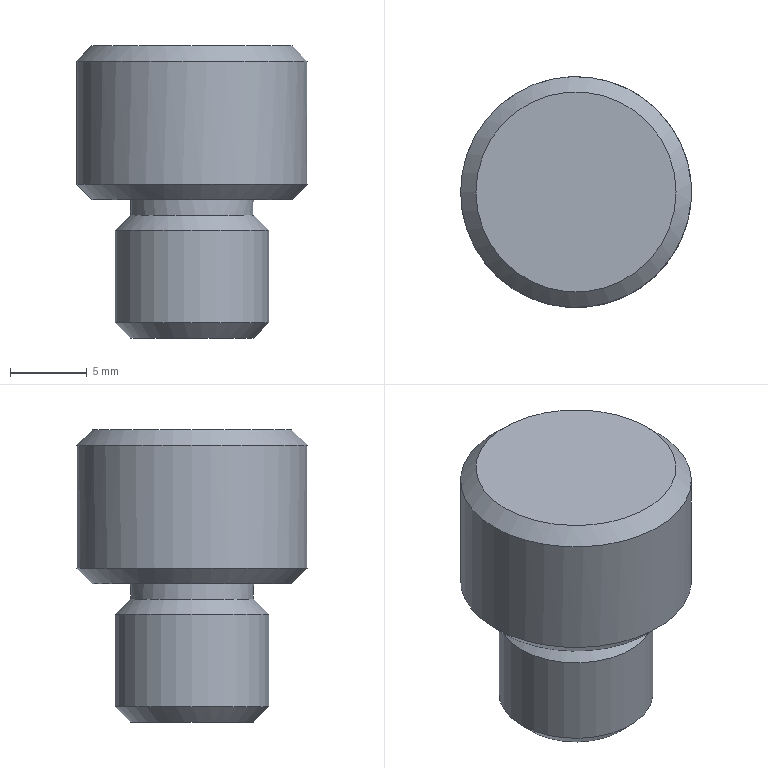Component | NX | SUPPORT_PIN | 1 solid | 10 faces | box 15 x 15 x 19 mm | volume 2371 mm3 | cone 4 | plane 3 | cylinder 3 | commonest cylinder face diameters 10 x1 8 x1 15 x1
STEP:
#1=CARTESIAN_POINT('',(0.,0.,0.));
#2=DIRECTION('',(0.,0.,1.));
#3=DIRECTION('',(1.,0.,0.));
#4=AXIS2_PLACEMENT_3D('',#1,#2,#3);
#5=CARTESIAN_POINT('',(-68.5,126.,81.));
#6=VERTEX_POINT('',#5);
#7=CARTESIAN_POINT('',(-72.5,126.,81.));
#8=DIRECTION('',(0.,0.,-1.));
#9=DIRECTION('',(1.,0.,0.));
#10=AXIS2_PLACEMENT_3D('',#7,#8,#9);
#11=CIRCLE('',#10,4.);
#12=CARTESIAN_POINT('',(-72.5,126.,81.));
#13=DIRECTION('',(0.,0.,-1.));
#14=DIRECTION('',(1.,0.,0.));
#15=AXIS2_PLACEMENT_3D('',#12,#13,#14);
#16=PLANE('',#15);
#17=CARTESIAN_POINT('',(0.,0.));
#18=DIRECTION('',(1.,0.));
#19=AXIS2_PLACEMENT_2D('',#17,#18);
#20=CIRCLE('',#19,4.);
#21=(GEOMETRIC_REPRESENTATION_CONTEXT(2)PARAMETRIC_REPRESENTATION_CONTEXT()REPRESENTATION_CONTEXT('',''));
#22=DEFINITIONAL_REPRESENTATION('',(#20),#21);
#23=PCURVE('',#16,#22);
#24=CARTESIAN_POINT('',(-72.5,126.,82.));
#25=DIRECTION('',(0.,0.,1.));
#26=DIRECTION('',(-1.,0.,0.));
#27=AXIS2_PLACEMENT_3D('',#24,#25,#26);
#28=CONICAL_SURFACE('',#27,5.,0.7854);
#29=CARTESIAN_POINT('',(9.425,-1.));
#30=DIRECTION('',(-1.,0.));
#31=VECTOR('',#30,1.);
#32=LINE('',#29,#31);
#33=(GEOMETRIC_REPRESENTATION_CONTEXT(2)PARAMETRIC_REPRESENTATION_CONTEXT()REPRESENTATION_CONTEXT('',''));
#34=DEFINITIONAL_REPRESENTATION('',(#32),#33);
#35=PCURVE('',#28,#34);
#36=SURFACE_CURVE('',#11,(#23,#35),.PCURVE_S1.);
#37=EDGE_CURVE('',#6,#6,#36,.T.);
#38=ORIENTED_EDGE('',*,*,#37,.T.);
#39=EDGE_LOOP('',(#38));
#40=FACE_BOUND('',#39,.T.);
#41=ADVANCED_FACE('',(#40),#16,.T.);
#42=CARTESIAN_POINT('',(-67.5,126.,82.));
#43=VERTEX_POINT('',#42);
#44=CARTESIAN_POINT('',(-77.5,126.,82.));
#45=VERTEX_POINT('',#44);
#46=CARTESIAN_POINT('',(-72.5,126.,82.));
#47=DIRECTION('',(0.,0.,1.));
#48=DIRECTION('',(1.,0.,0.));
#49=AXIS2_PLACEMENT_3D('',#46,#47,#48);
#50=CIRCLE('',#49,5.);
#51=CARTESIAN_POINT('',(-72.5,126.,81.));
#52=DIRECTION('',(0.,0.,1.));
#53=DIRECTION('',(-1.,0.,0.));
#54=AXIS2_PLACEMENT_3D('',#51,#52,#53);
#55=CYLINDRICAL_SURFACE('',#54,5.);
#56=CARTESIAN_POINT('',(3.142,1.));
#57=DIRECTION('',(1.,0.));
#58=VECTOR('',#57,1.);
#59=LINE('',#56,#58);
#60=(GEOMETRIC_REPRESENTATION_CONTEXT(2)PARAMETRIC_REPRESENTATION_CONTEXT()REPRESENTATION_CONTEXT('',''));
#61=DEFINITIONAL_REPRESENTATION('',(#59),#60);
#62=PCURVE('',#55,#61);
#63=CARTESIAN_POINT('',(3.142,0.));
#64=DIRECTION('',(1.,0.));
#65=VECTOR('',#64,1.);
#66=LINE('',#63,#65);
#67=(GEOMETRIC_REPRESENTATION_CONTEXT(2)PARAMETRIC_REPRESENTATION_CONTEXT()REPRESENTATION_CONTEXT('',''));
#68=DEFINITIONAL_REPRESENTATION('',(#66),#67);
#69=PCURVE('',#28,#68);
#70=SURFACE_CURVE('',#50,(#62,#69),.PCURVE_S1.);
#71=EDGE_CURVE('',#43,#45,#70,.T.);
#72=ORIENTED_EDGE('',*,*,#71,.T.);
#73=CARTESIAN_POINT('',(-77.5,126.,88.));
#74=VERTEX_POINT('',#73);
#75=CARTESIAN_POINT('',(-77.5,126.,82.));
#76=CARTESIAN_POINT('',(-77.5,126.,88.));
#77=B_SPLINE_CURVE_WITH_KNOTS('',1,(#75,#76),.UNSPECIFIED.,.F.,.F.,(2,2),(1.,7.),.PIECEWISE_BEZIER_KNOTS.);
#78=CARTESIAN_POINT('',(6.283,0.));
#79=DIRECTION('',(0.,1.));
#80=VECTOR('',#79,1.);
#81=LINE('',#78,#80);
#82=(GEOMETRIC_REPRESENTATION_CONTEXT(2)PARAMETRIC_REPRESENTATION_CONTEXT()REPRESENTATION_CONTEXT('',''));
#83=DEFINITIONAL_REPRESENTATION('',(#81),#82);
#84=PCURVE('',#55,#83);
#85=CARTESIAN_POINT('',(0.,0.));
#86=DIRECTION('',(0.,1.));
#87=VECTOR('',#86,1.);
#88=LINE('',#85,#87);
#89=(GEOMETRIC_REPRESENTATION_CONTEXT(2)PARAMETRIC_REPRESENTATION_CONTEXT()REPRESENTATION_CONTEXT('',''));
#90=DEFINITIONAL_REPRESENTATION('',(#88),#89);
#91=PCURVE('',#55,#90);
#92=SEAM_CURVE('',#77,(#84,#91),.PCURVE_S1.);
#93=EDGE_CURVE('',#45,#74,#92,.T.);
#94=ORIENTED_EDGE('',*,*,#93,.T.);
#95=CARTESIAN_POINT('',(-72.5,126.,88.));
#96=DIRECTION('',(0.,0.,-1.));
#97=DIRECTION('',(-1.,0.,0.));
#98=AXIS2_PLACEMENT_3D('',#95,#96,#97);
#99=CIRCLE('',#98,5.);
#100=CARTESIAN_POINT('',(6.283,7.));
#101=DIRECTION('',(-1.,0.));
#102=VECTOR('',#101,1.);
#103=LINE('',#100,#102);
#104=(GEOMETRIC_REPRESENTATION_CONTEXT(2)PARAMETRIC_REPRESENTATION_CONTEXT()REPRESENTATION_CONTEXT('',''));
#105=DEFINITIONAL_REPRESENTATION('',(#103),#104);
#106=PCURVE('',#55,#105);
#107=CARTESIAN_POINT('',(-72.5,126.,88.));
#108=DIRECTION('',(0.,0.,-1.));
#109=DIRECTION('',(1.,0.,0.));
#110=AXIS2_PLACEMENT_3D('',#107,#108,#109);
#111=CONICAL_SURFACE('',#110,5.,0.7854);
#112=CARTESIAN_POINT('',(3.142,0.));
#113=DIRECTION('',(1.,0.));
#114=VECTOR('',#113,1.);
#115=LINE('',#112,#114);
#116=(GEOMETRIC_REPRESENTATION_CONTEXT(2)PARAMETRIC_REPRESENTATION_CONTEXT()REPRESENTATION_CONTEXT('',''));
#117=DEFINITIONAL_REPRESENTATION('',(#115),#116);
#118=PCURVE('',#111,#117);
#119=SURFACE_CURVE('',#99,(#106,#118),.PCURVE_S1.);
#120=EDGE_CURVE('',#74,#74,#119,.T.);
#121=ORIENTED_EDGE('',*,*,#120,.T.);
#122=ORIENTED_EDGE('',*,*,#93,.F.);
#123=CARTESIAN_POINT('',(-72.5,126.,82.));
#124=DIRECTION('',(0.,0.,1.));
#125=DIRECTION('',(1.,0.,0.));
#126=AXIS2_PLACEMENT_3D('',#123,#124,#125);
#127=CIRCLE('',#126,5.);
#128=CARTESIAN_POINT('',(-3.142,1.));
#129=DIRECTION('',(1.,0.));
#130=VECTOR('',#129,1.);
#131=LINE('',#128,#130);
#132=(GEOMETRIC_REPRESENTATION_CONTEXT(2)PARAMETRIC_REPRESENTATION_CONTEXT()REPRESENTATION_CONTEXT('',''));
#133=DEFINITIONAL_REPRESENTATION('',(#131),#132);
#134=PCURVE('',#55,#133);
#135=CARTESIAN_POINT('',(3.142,0.));
#136=DIRECTION('',(1.,0.));
#137=VECTOR('',#136,1.);
#138=LINE('',#135,#137);
#139=(GEOMETRIC_REPRESENTATION_CONTEXT(2)PARAMETRIC_REPRESENTATION_CONTEXT()REPRESENTATION_CONTEXT('',''));
#140=DEFINITIONAL_REPRESENTATION('',(#138),#139);
#141=PCURVE('',#28,#140);
#142=SURFACE_CURVE('',#127,(#134,#141),.PCURVE_S1.);
#143=EDGE_CURVE('',#45,#43,#142,.T.);
#144=ORIENTED_EDGE('',*,*,#143,.T.);
#145=EDGE_LOOP('',(#72,#94,#121,#122,#144));
#146=FACE_BOUND('',#145,.T.);
#147=ADVANCED_FACE('',(#146),#55,.T.);
#148=CARTESIAN_POINT('',(-76.5,126.,90.));
#149=VERTEX_POINT('',#148);
#150=CARTESIAN_POINT('',(-68.5,126.,90.));
#151=VERTEX_POINT('',#150);
#152=CARTESIAN_POINT('',(-72.5,126.,90.));
#153=DIRECTION('',(0.,0.,1.));
#154=DIRECTION('',(1.,0.,0.));
#155=AXIS2_PLACEMENT_3D('',#152,#153,#154);
#156=CIRCLE('',#155,4.);
#157=CARTESIAN_POINT('',(-72.5,126.,89.));
#158=DIRECTION('',(0.,0.,1.));
#159=DIRECTION('',(-1.,0.,0.));
#160=AXIS2_PLACEMENT_3D('',#157,#158,#159);
#161=CYLINDRICAL_SURFACE('',#160,4.);
#162=CARTESIAN_POINT('',(-3.142,1.));
#163=DIRECTION('',(1.,0.));
#164=VECTOR('',#163,1.);
#165=LINE('',#162,#164);
#166=(GEOMETRIC_REPRESENTATION_CONTEXT(2)PARAMETRIC_REPRESENTATION_CONTEXT()REPRESENTATION_CONTEXT('',''));
#167=DEFINITIONAL_REPRESENTATION('',(#165),#166);
#168=PCURVE('',#161,#167);
#169=CARTESIAN_POINT('',(-72.5,126.,90.));
#170=DIRECTION('',(0.,0.,-1.));
#171=DIRECTION('',(1.,0.,0.));
#172=AXIS2_PLACEMENT_3D('',#169,#170,#171);
#173=PLANE('',#172);
#174=CARTESIAN_POINT('',(4.,0.));
#175=CARTESIAN_POINT('',(4.,-6.928));
#176=CARTESIAN_POINT('',(-2.,-3.464));
#177=CARTESIAN_POINT('',(-8.,-0.));
#178=CARTESIAN_POINT('',(-2.,3.464));
#179=CARTESIAN_POINT('',(4.,6.928));
#180=CARTESIAN_POINT('',(4.,0.));
#181=(BOUNDED_CURVE()B_SPLINE_CURVE(2,(#174,#175,#176,#177,#178,#179,#180),.UNSPECIFIED.,.T.,.F.)B_SPLINE_CURVE_WITH_KNOTS((1,2,2,2,2,1),(-2.094,0.,2.094,4.189,6.283,8.378),.UNSPECIFIED.)CURVE()GEOMETRIC_REPRESENTATION_ITEM()RATIONAL_B_SPLINE_CURVE((1.,0.5,1.,0.5,1.,0.5,1.))REPRESENTATION_ITEM(''));
#182=(GEOMETRIC_REPRESENTATION_CONTEXT(2)PARAMETRIC_REPRESENTATION_CONTEXT()REPRESENTATION_CONTEXT('',''));
#183=DEFINITIONAL_REPRESENTATION('',(#181),#182);
#184=PCURVE('',#173,#183);
#185=SURFACE_CURVE('',#156,(#168,#184),.PCURVE_S1.);
#186=EDGE_CURVE('',#149,#151,#185,.T.);
#187=ORIENTED_EDGE('',*,*,#186,.F.);
#188=CARTESIAN_POINT('',(-76.5,126.,89.));
#189=VERTEX_POINT('',#188);
#190=CARTESIAN_POINT('',(-76.5,126.,89.));
#191=CARTESIAN_POINT('',(-76.5,126.,90.));
#192=B_SPLINE_CURVE_WITH_KNOTS('',1,(#190,#191),.UNSPECIFIED.,.F.,.F.,(2,2),(0.,1.),.PIECEWISE_BEZIER_KNOTS.);
#193=CARTESIAN_POINT('',(0.,0.));
#194=DIRECTION('',(0.,1.));
#195=VECTOR('',#194,1.);
#196=LINE('',#193,#195);
#197=(GEOMETRIC_REPRESENTATION_CONTEXT(2)PARAMETRIC_REPRESENTATION_CONTEXT()REPRESENTATION_CONTEXT('',''));
#198=DEFINITIONAL_REPRESENTATION('',(#196),#197);
#199=PCURVE('',#161,#198);
#200=CARTESIAN_POINT('',(6.283,0.));
#201=DIRECTION('',(0.,1.));
#202=VECTOR('',#201,1.);
#203=LINE('',#200,#202);
#204=(GEOMETRIC_REPRESENTATION_CONTEXT(2)PARAMETRIC_REPRESENTATION_CONTEXT()REPRESENTATION_CONTEXT('',''));
#205=DEFINITIONAL_REPRESENTATION('',(#203),#204);
#206=PCURVE('',#161,#205);
#207=SEAM_CURVE('',#192,(#199,#206),.PCURVE_S1.);
#208=EDGE_CURVE('',#189,#149,#207,.T.);
#209=ORIENTED_EDGE('',*,*,#208,.F.);
#210=CARTESIAN_POINT('',(-72.5,126.,89.));
#211=DIRECTION('',(0.,0.,1.));
#212=DIRECTION('',(-1.,0.,0.));
#213=AXIS2_PLACEMENT_3D('',#210,#211,#212);
#214=CIRCLE('',#213,4.);
#215=CARTESIAN_POINT('',(0.,0.));
#216=DIRECTION('',(1.,0.));
#217=VECTOR('',#216,1.);
#218=LINE('',#215,#217);
#219=(GEOMETRIC_REPRESENTATION_CONTEXT(2)PARAMETRIC_REPRESENTATION_CONTEXT()REPRESENTATION_CONTEXT('',''));
#220=DEFINITIONAL_REPRESENTATION('',(#218),#219);
#221=PCURVE('',#161,#220);
#222=CARTESIAN_POINT('',(9.425,-1.));
#223=DIRECTION('',(-1.,0.));
#224=VECTOR('',#223,1.);
#225=LINE('',#222,#224);
#226=(GEOMETRIC_REPRESENTATION_CONTEXT(2)PARAMETRIC_REPRESENTATION_CONTEXT()REPRESENTATION_CONTEXT('',''));
#227=DEFINITIONAL_REPRESENTATION('',(#225),#226);
#228=PCURVE('',#111,#227);
#229=SURFACE_CURVE('',#214,(#221,#228),.PCURVE_S1.);
#230=EDGE_CURVE('',#189,#189,#229,.T.);
#231=ORIENTED_EDGE('',*,*,#230,.T.);
#232=ORIENTED_EDGE('',*,*,#208,.T.);
#233=CARTESIAN_POINT('',(-72.5,126.,90.));
#234=DIRECTION('',(0.,0.,1.));
#235=DIRECTION('',(1.,0.,0.));
#236=AXIS2_PLACEMENT_3D('',#233,#234,#235);
#237=CIRCLE('',#236,4.);
#238=CARTESIAN_POINT('',(3.142,1.));
#239=DIRECTION('',(1.,0.));
#240=VECTOR('',#239,1.);
#241=LINE('',#238,#240);
#242=(GEOMETRIC_REPRESENTATION_CONTEXT(2)PARAMETRIC_REPRESENTATION_CONTEXT()REPRESENTATION_CONTEXT('',''));
#243=DEFINITIONAL_REPRESENTATION('',(#241),#242);
#244=PCURVE('',#161,#243);
#245=CARTESIAN_POINT('',(4.,0.));
#246=CARTESIAN_POINT('',(4.,-6.928));
#247=CARTESIAN_POINT('',(-2.,-3.464));
#248=CARTESIAN_POINT('',(-8.,-0.));
#249=CARTESIAN_POINT('',(-2.,3.464));
#250=CARTESIAN_POINT('',(4.,6.928));
#251=CARTESIAN_POINT('',(4.,0.));
#252=(BOUNDED_CURVE()B_SPLINE_CURVE(2,(#245,#246,#247,#248,#249,#250,#251),.UNSPECIFIED.,.T.,.F.)B_SPLINE_CURVE_WITH_KNOTS((1,2,2,2,2,1),(-2.094,0.,2.094,4.189,6.283,8.378),.UNSPECIFIED.)CURVE()GEOMETRIC_REPRESENTATION_ITEM()RATIONAL_B_SPLINE_CURVE((1.,0.5,1.,0.5,1.,0.5,1.))REPRESENTATION_ITEM(''));
#253=(GEOMETRIC_REPRESENTATION_CONTEXT(2)PARAMETRIC_REPRESENTATION_CONTEXT()REPRESENTATION_CONTEXT('',''));
#254=DEFINITIONAL_REPRESENTATION('',(#252),#253);
#255=PCURVE('',#173,#254);
#256=SURFACE_CURVE('',#237,(#244,#255),.PCURVE_S1.);
#257=EDGE_CURVE('',#151,#149,#256,.T.);
#258=ORIENTED_EDGE('',*,*,#257,.F.);
#259=EDGE_LOOP('',(#187,#209,#231,#232,#258));
#260=FACE_BOUND('',#259,.T.);
#261=ADVANCED_FACE('',(#260),#161,.T.);
#262=CARTESIAN_POINT('',(-79.,126.,100.));
#263=VERTEX_POINT('',#262);
#264=CARTESIAN_POINT('',(-72.5,126.,100.));
#265=DIRECTION('',(0.,0.,1.));
#266=DIRECTION('',(-1.,0.,0.));
#267=AXIS2_PLACEMENT_3D('',#264,#265,#266);
#268=CIRCLE('',#267,6.5);
#269=CARTESIAN_POINT('',(-72.5,126.,100.));
#270=DIRECTION('',(0.,0.,1.));
#271=DIRECTION('',(-1.,0.,0.));
#272=AXIS2_PLACEMENT_3D('',#269,#270,#271);
#273=PLANE('',#272);
#274=CARTESIAN_POINT('',(0.,0.));
#275=DIRECTION('',(1.,0.));
#276=AXIS2_PLACEMENT_2D('',#274,#275);
#277=CIRCLE('',#276,6.5);
#278=(GEOMETRIC_REPRESENTATION_CONTEXT(2)PARAMETRIC_REPRESENTATION_CONTEXT()REPRESENTATION_CONTEXT('',''));
#279=DEFINITIONAL_REPRESENTATION('',(#277),#278);
#280=PCURVE('',#273,#279);
#281=CARTESIAN_POINT('',(-72.5,126.,99.));
#282=DIRECTION('',(0.,0.,-1.));
#283=DIRECTION('',(1.,0.,0.));
#284=AXIS2_PLACEMENT_3D('',#281,#282,#283);
#285=CONICAL_SURFACE('',#284,7.5,0.7854);
#286=CARTESIAN_POINT('',(9.425,-1.));
#287=DIRECTION('',(-1.,0.));
#288=VECTOR('',#287,1.);
#289=LINE('',#286,#288);
#290=(GEOMETRIC_REPRESENTATION_CONTEXT(2)PARAMETRIC_REPRESENTATION_CONTEXT()REPRESENTATION_CONTEXT('',''));
#291=DEFINITIONAL_REPRESENTATION('',(#289),#290);
#292=PCURVE('',#285,#291);
#293=SURFACE_CURVE('',#268,(#280,#292),.PCURVE_S1.);
#294=EDGE_CURVE('',#263,#263,#293,.T.);
#295=ORIENTED_EDGE('',*,*,#294,.T.);
#296=EDGE_LOOP('',(#295));
#297=FACE_BOUND('',#296,.T.);
#298=ADVANCED_FACE('',(#297),#273,.T.);
#299=CARTESIAN_POINT('',(-66.,126.,90.));
#300=VERTEX_POINT('',#299);
#301=CARTESIAN_POINT('',(-72.5,126.,90.));
#302=DIRECTION('',(0.,0.,-1.));
#303=DIRECTION('',(1.,0.,0.));
#304=AXIS2_PLACEMENT_3D('',#301,#302,#303);
#305=CIRCLE('',#304,6.5);
#306=CARTESIAN_POINT('',(0.,0.));
#307=DIRECTION('',(1.,0.));
#308=AXIS2_PLACEMENT_2D('',#306,#307);
#309=CIRCLE('',#308,6.5);
#310=(GEOMETRIC_REPRESENTATION_CONTEXT(2)PARAMETRIC_REPRESENTATION_CONTEXT()REPRESENTATION_CONTEXT('',''));
#311=DEFINITIONAL_REPRESENTATION('',(#309),#310);
#312=PCURVE('',#173,#311);
#313=CARTESIAN_POINT('',(-72.5,126.,91.));
#314=DIRECTION('',(0.,0.,1.));
#315=DIRECTION('',(-1.,0.,0.));
#316=AXIS2_PLACEMENT_3D('',#313,#314,#315);
#317=CONICAL_SURFACE('',#316,7.5,0.7854);
#318=CARTESIAN_POINT('',(9.425,-1.));
#319=DIRECTION('',(-1.,0.));
#320=VECTOR('',#319,1.);
#321=LINE('',#318,#320);
#322=(GEOMETRIC_REPRESENTATION_CONTEXT(2)PARAMETRIC_REPRESENTATION_CONTEXT()REPRESENTATION_CONTEXT('',''));
#323=DEFINITIONAL_REPRESENTATION('',(#321),#322);
#324=PCURVE('',#317,#323);
#325=SURFACE_CURVE('',#305,(#312,#324),.PCURVE_S1.);
#326=EDGE_CURVE('',#300,#300,#325,.T.);
#327=ORIENTED_EDGE('',*,*,#326,.T.);
#328=EDGE_LOOP('',(#327));
#329=FACE_BOUND('',#328,.T.);
#330=ORIENTED_EDGE('',*,*,#257,.T.);
#331=ORIENTED_EDGE('',*,*,#186,.T.);
#332=EDGE_LOOP('',(#330,#331));
#333=FACE_BOUND('',#332,.T.);
#334=ADVANCED_FACE('',(#329,#333),#173,.T.);
#335=CARTESIAN_POINT('',(-65.,126.,91.));
#336=VERTEX_POINT('',#335);
#337=CARTESIAN_POINT('',(-80.,126.,91.));
#338=VERTEX_POINT('',#337);
#339=CARTESIAN_POINT('',(-72.5,126.,91.));
#340=DIRECTION('',(0.,0.,1.));
#341=DIRECTION('',(1.,0.,0.));
#342=AXIS2_PLACEMENT_3D('',#339,#340,#341);
#343=CIRCLE('',#342,7.5);
#344=CARTESIAN_POINT('',(-72.5,126.,90.));
#345=DIRECTION('',(0.,0.,1.));
#346=DIRECTION('',(-1.,0.,0.));
#347=AXIS2_PLACEMENT_3D('',#344,#345,#346);
#348=CYLINDRICAL_SURFACE('',#347,7.5);
#349=CARTESIAN_POINT('',(3.142,1.));
#350=DIRECTION('',(1.,0.));
#351=VECTOR('',#350,1.);
#352=LINE('',#349,#351);
#353=(GEOMETRIC_REPRESENTATION_CONTEXT(2)PARAMETRIC_REPRESENTATION_CONTEXT()REPRESENTATION_CONTEXT('',''));
#354=DEFINITIONAL_REPRESENTATION('',(#352),#353);
#355=PCURVE('',#348,#354);
#356=CARTESIAN_POINT('',(3.142,0.));
#357=DIRECTION('',(1.,0.));
#358=VECTOR('',#357,1.);
#359=LINE('',#356,#358);
#360=(GEOMETRIC_REPRESENTATION_CONTEXT(2)PARAMETRIC_REPRESENTATION_CONTEXT()REPRESENTATION_CONTEXT('',''));
#361=DEFINITIONAL_REPRESENTATION('',(#359),#360);
#362=PCURVE('',#317,#361);
#363=SURFACE_CURVE('',#343,(#355,#362),.PCURVE_S1.);
#364=EDGE_CURVE('',#336,#338,#363,.T.);
#365=ORIENTED_EDGE('',*,*,#364,.T.);
#366=CARTESIAN_POINT('',(-80.,126.,99.));
#367=VERTEX_POINT('',#366);
#368=CARTESIAN_POINT('',(-80.,126.,91.));
#369=CARTESIAN_POINT('',(-80.,126.,99.));
#370=B_SPLINE_CURVE_WITH_KNOTS('',1,(#368,#369),.UNSPECIFIED.,.F.,.F.,(2,2),(1.,9.),.PIECEWISE_BEZIER_KNOTS.);
#371=CARTESIAN_POINT('',(6.283,0.));
#372=DIRECTION('',(0.,1.));
#373=VECTOR('',#372,1.);
#374=LINE('',#371,#373);
#375=(GEOMETRIC_REPRESENTATION_CONTEXT(2)PARAMETRIC_REPRESENTATION_CONTEXT()REPRESENTATION_CONTEXT('',''));
#376=DEFINITIONAL_REPRESENTATION('',(#374),#375);
#377=PCURVE('',#348,#376);
#378=CARTESIAN_POINT('',(0.,0.));
#379=DIRECTION('',(0.,1.));
#380=VECTOR('',#379,1.);
#381=LINE('',#378,#380);
#382=(GEOMETRIC_REPRESENTATION_CONTEXT(2)PARAMETRIC_REPRESENTATION_CONTEXT()REPRESENTATION_CONTEXT('',''));
#383=DEFINITIONAL_REPRESENTATION('',(#381),#382);
#384=PCURVE('',#348,#383);
#385=SEAM_CURVE('',#370,(#377,#384),.PCURVE_S1.);
#386=EDGE_CURVE('',#338,#367,#385,.T.);
#387=ORIENTED_EDGE('',*,*,#386,.T.);
#388=CARTESIAN_POINT('',(-72.5,126.,99.));
#389=DIRECTION('',(0.,0.,-1.));
#390=DIRECTION('',(-1.,0.,0.));
#391=AXIS2_PLACEMENT_3D('',#388,#389,#390);
#392=CIRCLE('',#391,7.5);
#393=CARTESIAN_POINT('',(6.283,9.));
#394=DIRECTION('',(-1.,0.));
#395=VECTOR('',#394,1.);
#396=LINE('',#393,#395);
#397=(GEOMETRIC_REPRESENTATION_CONTEXT(2)PARAMETRIC_REPRESENTATION_CONTEXT()REPRESENTATION_CONTEXT('',''));
#398=DEFINITIONAL_REPRESENTATION('',(#396),#397);
#399=PCURVE('',#348,#398);
#400=CARTESIAN_POINT('',(3.142,0.));
#401=DIRECTION('',(1.,0.));
#402=VECTOR('',#401,1.);
#403=LINE('',#400,#402);
#404=(GEOMETRIC_REPRESENTATION_CONTEXT(2)PARAMETRIC_REPRESENTATION_CONTEXT()REPRESENTATION_CONTEXT('',''));
#405=DEFINITIONAL_REPRESENTATION('',(#403),#404);
#406=PCURVE('',#285,#405);
#407=SURFACE_CURVE('',#392,(#399,#406),.PCURVE_S1.);
#408=EDGE_CURVE('',#367,#367,#407,.T.);
#409=ORIENTED_EDGE('',*,*,#408,.T.);
#410=ORIENTED_EDGE('',*,*,#386,.F.);
#411=CARTESIAN_POINT('',(-72.5,126.,91.));
#412=DIRECTION('',(0.,0.,1.));
#413=DIRECTION('',(1.,0.,0.));
#414=AXIS2_PLACEMENT_3D('',#411,#412,#413);
#415=CIRCLE('',#414,7.5);
#416=CARTESIAN_POINT('',(-3.142,1.));
#417=DIRECTION('',(1.,0.));
#418=VECTOR('',#417,1.);
#419=LINE('',#416,#418);
#420=(GEOMETRIC_REPRESENTATION_CONTEXT(2)PARAMETRIC_REPRESENTATION_CONTEXT()REPRESENTATION_CONTEXT('',''));
#421=DEFINITIONAL_REPRESENTATION('',(#419),#420);
#422=PCURVE('',#348,#421);
#423=CARTESIAN_POINT('',(3.142,0.));
#424=DIRECTION('',(1.,0.));
#425=VECTOR('',#424,1.);
#426=LINE('',#423,#425);
#427=(GEOMETRIC_REPRESENTATION_CONTEXT(2)PARAMETRIC_REPRESENTATION_CONTEXT()REPRESENTATION_CONTEXT('',''));
#428=DEFINITIONAL_REPRESENTATION('',(#426),#427);
#429=PCURVE('',#317,#428);
#430=SURFACE_CURVE('',#415,(#422,#429),.PCURVE_S1.);
#431=EDGE_CURVE('',#338,#336,#430,.T.);
#432=ORIENTED_EDGE('',*,*,#431,.T.);
#433=EDGE_LOOP('',(#365,#387,#409,#410,#432));
#434=FACE_BOUND('',#433,.T.);
#435=ADVANCED_FACE('',(#434),#348,.T.);
#436=ORIENTED_EDGE('',*,*,#37,.F.);
#437=CARTESIAN_POINT('',(-68.5,126.,81.));
#438=CARTESIAN_POINT('',(-67.5,126.,82.));
#439=B_SPLINE_CURVE_WITH_KNOTS('',1,(#437,#438),.UNSPECIFIED.,.F.,.F.,(2,2),(-1.414,0.),.PIECEWISE_BEZIER_KNOTS.);
#440=CARTESIAN_POINT('',(9.425,0.));
#441=DIRECTION('',(0.,1.));
#442=VECTOR('',#441,1.);
#443=LINE('',#440,#442);
#444=(GEOMETRIC_REPRESENTATION_CONTEXT(2)PARAMETRIC_REPRESENTATION_CONTEXT()REPRESENTATION_CONTEXT('',''));
#445=DEFINITIONAL_REPRESENTATION('',(#443),#444);
#446=PCURVE('',#28,#445);
#447=CARTESIAN_POINT('',(3.142,0.));
#448=DIRECTION('',(0.,1.));
#449=VECTOR('',#448,1.);
#450=LINE('',#447,#449);
#451=(GEOMETRIC_REPRESENTATION_CONTEXT(2)PARAMETRIC_REPRESENTATION_CONTEXT()REPRESENTATION_CONTEXT('',''));
#452=DEFINITIONAL_REPRESENTATION('',(#450),#451);
#453=PCURVE('',#28,#452);
#454=SEAM_CURVE('',#439,(#446,#453),.PCURVE_S1.);
#455=EDGE_CURVE('',#6,#43,#454,.T.);
#456=ORIENTED_EDGE('',*,*,#455,.T.);
#457=ORIENTED_EDGE('',*,*,#143,.F.);
#458=ORIENTED_EDGE('',*,*,#71,.F.);
#459=ORIENTED_EDGE('',*,*,#455,.F.);
#460=EDGE_LOOP('',(#436,#456,#457,#458,#459));
#461=FACE_BOUND('',#460,.T.);
#462=ADVANCED_FACE('',(#461),#28,.T.);
#463=ORIENTED_EDGE('',*,*,#230,.F.);
#464=CARTESIAN_POINT('',(-76.5,126.,89.));
#465=CARTESIAN_POINT('',(-77.5,126.,88.));
#466=B_SPLINE_CURVE_WITH_KNOTS('',1,(#464,#465),.UNSPECIFIED.,.F.,.F.,(2,2),(-1.414,0.),.PIECEWISE_BEZIER_KNOTS.);
#467=CARTESIAN_POINT('',(9.425,0.));
#468=DIRECTION('',(0.,1.));
#469=VECTOR('',#468,1.);
#470=LINE('',#467,#469);
#471=(GEOMETRIC_REPRESENTATION_CONTEXT(2)PARAMETRIC_REPRESENTATION_CONTEXT()REPRESENTATION_CONTEXT('',''));
#472=DEFINITIONAL_REPRESENTATION('',(#470),#471);
#473=PCURVE('',#111,#472);
#474=CARTESIAN_POINT('',(3.142,0.));
#475=DIRECTION('',(0.,1.));
#476=VECTOR('',#475,1.);
#477=LINE('',#474,#476);
#478=(GEOMETRIC_REPRESENTATION_CONTEXT(2)PARAMETRIC_REPRESENTATION_CONTEXT()REPRESENTATION_CONTEXT('',''));
#479=DEFINITIONAL_REPRESENTATION('',(#477),#478);
#480=PCURVE('',#111,#479);
#481=SEAM_CURVE('',#466,(#473,#480),.PCURVE_S1.);
#482=EDGE_CURVE('',#189,#74,#481,.T.);
#483=ORIENTED_EDGE('',*,*,#482,.T.);
#484=ORIENTED_EDGE('',*,*,#120,.F.);
#485=ORIENTED_EDGE('',*,*,#482,.F.);
#486=EDGE_LOOP('',(#463,#483,#484,#485));
#487=FACE_BOUND('',#486,.T.);
#488=ADVANCED_FACE('',(#487),#111,.T.);
#489=ORIENTED_EDGE('',*,*,#326,.F.);
#490=CARTESIAN_POINT('',(-66.,126.,90.));
#491=CARTESIAN_POINT('',(-65.,126.,91.));
#492=B_SPLINE_CURVE_WITH_KNOTS('',1,(#490,#491),.UNSPECIFIED.,.F.,.F.,(2,2),(-1.414,0.),.PIECEWISE_BEZIER_KNOTS.);
#493=CARTESIAN_POINT('',(9.425,0.));
#494=DIRECTION('',(0.,1.));
#495=VECTOR('',#494,1.);
#496=LINE('',#493,#495);
#497=(GEOMETRIC_REPRESENTATION_CONTEXT(2)PARAMETRIC_REPRESENTATION_CONTEXT()REPRESENTATION_CONTEXT('',''));
#498=DEFINITIONAL_REPRESENTATION('',(#496),#497);
#499=PCURVE('',#317,#498);
#500=CARTESIAN_POINT('',(3.142,0.));
#501=DIRECTION('',(0.,1.));
#502=VECTOR('',#501,1.);
#503=LINE('',#500,#502);
#504=(GEOMETRIC_REPRESENTATION_CONTEXT(2)PARAMETRIC_REPRESENTATION_CONTEXT()REPRESENTATION_CONTEXT('',''));
#505=DEFINITIONAL_REPRESENTATION('',(#503),#504);
#506=PCURVE('',#317,#505);
#507=SEAM_CURVE('',#492,(#499,#506),.PCURVE_S1.);
#508=EDGE_CURVE('',#300,#336,#507,.T.);
#509=ORIENTED_EDGE('',*,*,#508,.T.);
#510=ORIENTED_EDGE('',*,*,#431,.F.);
#511=ORIENTED_EDGE('',*,*,#364,.F.);
#512=ORIENTED_EDGE('',*,*,#508,.F.);
#513=EDGE_LOOP('',(#489,#509,#510,#511,#512));
#514=FACE_BOUND('',#513,.T.);
#515=ADVANCED_FACE('',(#514),#317,.T.);
#516=ORIENTED_EDGE('',*,*,#294,.F.);
#517=CARTESIAN_POINT('',(-79.,126.,100.));
#518=CARTESIAN_POINT('',(-80.,126.,99.));
#519=B_SPLINE_CURVE_WITH_KNOTS('',1,(#517,#518),.UNSPECIFIED.,.F.,.F.,(2,2),(-1.414,0.),.PIECEWISE_BEZIER_KNOTS.);
#520=CARTESIAN_POINT('',(9.425,0.));
#521=DIRECTION('',(0.,1.));
#522=VECTOR('',#521,1.);
#523=LINE('',#520,#522);
#524=(GEOMETRIC_REPRESENTATION_CONTEXT(2)PARAMETRIC_REPRESENTATION_CONTEXT()REPRESENTATION_CONTEXT('',''));
#525=DEFINITIONAL_REPRESENTATION('',(#523),#524);
#526=PCURVE('',#285,#525);
#527=CARTESIAN_POINT('',(3.142,0.));
#528=DIRECTION('',(0.,1.));
#529=VECTOR('',#528,1.);
#530=LINE('',#527,#529);
#531=(GEOMETRIC_REPRESENTATION_CONTEXT(2)PARAMETRIC_REPRESENTATION_CONTEXT()REPRESENTATION_CONTEXT('',''));
#532=DEFINITIONAL_REPRESENTATION('',(#530),#531);
#533=PCURVE('',#285,#532);
#534=SEAM_CURVE('',#519,(#526,#533),.PCURVE_S1.);
#535=EDGE_CURVE('',#263,#367,#534,.T.);
#536=ORIENTED_EDGE('',*,*,#535,.T.);
#537=ORIENTED_EDGE('',*,*,#408,.F.);
#538=ORIENTED_EDGE('',*,*,#535,.F.);
#539=EDGE_LOOP('',(#516,#536,#537,#538));
#540=FACE_BOUND('',#539,.T.);
#541=ADVANCED_FACE('',(#540),#285,.T.);
#542=CLOSED_SHELL('',(#41,#147,#261,#298,#334,#435,#462,#488,#515,#541));
#543=MANIFOLD_SOLID_BREP('',#542);
#544=(LENGTH_UNIT()NAMED_UNIT(*)SI_UNIT(.MILLI.,.METRE.));
#545=UNCERTAINTY_MEASURE_WITH_UNIT(LENGTH_MEASURE(0.00001),#544,'','');
#546=(NAMED_UNIT(*)PLANE_ANGLE_UNIT()SI_UNIT($,.RADIAN.));
#547=(NAMED_UNIT(*)SI_UNIT($,.STERADIAN.)SOLID_ANGLE_UNIT());
#548=(GEOMETRIC_REPRESENTATION_CONTEXT(3)GLOBAL_UNCERTAINTY_ASSIGNED_CONTEXT((#545))GLOBAL_UNIT_ASSIGNED_CONTEXT((#544,#546,#547))REPRESENTATION_CONTEXT('',''));
#549=ADVANCED_BREP_SHAPE_REPRESENTATION('',(#4,#543),#548);